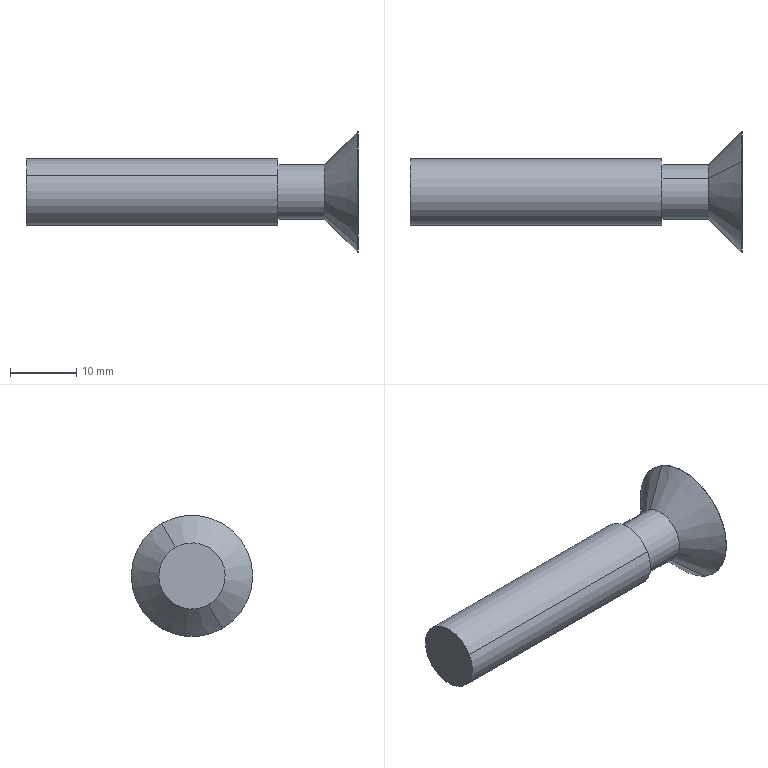Component | SolidWorks | CountersunkScrew-2 | 1 solid | 36 faces | box 50.07 x 18.3 x 18.3 mm | volume 3945 mm3 | plane 24 | cylinder 10 | cone 2 | commonest cylinder face diameters 4 x4 18.3 x2 8.3 x2 10 x2
STEP:
#1=COLOUR_RGB('',0.7922,0.8196,0.9333);
#2=FILL_AREA_STYLE_COLOUR('',#1);
#3=FILL_AREA_STYLE('',(#2));
#4=SURFACE_STYLE_FILL_AREA(#3);
#5=SURFACE_SIDE_STYLE('',(#4));
#6=SURFACE_STYLE_USAGE(.BOTH.,#5);
#7=PRESENTATION_STYLE_ASSIGNMENT((#6));
#8=CARTESIAN_POINT('',(2.939,29.846,46.096));
#9=VERTEX_POINT('',#8);
#10=CARTESIAN_POINT('',(2.939,30.206,46.72));
#11=VERTEX_POINT('',#10);
#12=CARTESIAN_POINT('',(2.939,30.026,46.408));
#13=DIRECTION('',(1.,0.,0.));
#14=DIRECTION('',(0.,-0.5,-0.866));
#15=AXIS2_PLACEMENT_3D('',#12,#13,#14);
#16=CIRCLE('',#15,0.3602);
#17=EDGE_CURVE('',#9,#11,#16,.T.);
#18=ORIENTED_EDGE('',*,*,#17,.F.);
#19=CARTESIAN_POINT('',(2.937,29.846,46.096));
#20=VERTEX_POINT('',#19);
#21=CARTESIAN_POINT('',(2.939,29.846,46.096));
#22=DIRECTION('',(-1.,0.,0.));
#23=VECTOR('',#22,39.37);
#24=LINE('',#21,#23);
#25=EDGE_CURVE('',#9,#20,#24,.T.);
#26=ORIENTED_EDGE('',*,*,#25,.T.);
#27=CARTESIAN_POINT('',(2.937,30.206,46.72));
#28=VERTEX_POINT('',#27);
#29=CARTESIAN_POINT('',(2.937,30.026,46.408));
#30=DIRECTION('',(1.,0.,0.));
#31=DIRECTION('',(0.,-0.5,-0.866));
#32=AXIS2_PLACEMENT_3D('',#29,#30,#31);
#33=CIRCLE('',#32,0.3602);
#34=EDGE_CURVE('',#20,#28,#33,.T.);
#35=ORIENTED_EDGE('',*,*,#34,.T.);
#36=CARTESIAN_POINT('',(2.939,30.206,46.72));
#37=DIRECTION('',(-1.,0.,0.));
#38=VECTOR('',#37,39.37);
#39=LINE('',#36,#38);
#40=EDGE_CURVE('',#11,#28,#39,.T.);
#41=ORIENTED_EDGE('',*,*,#40,.F.);
#42=EDGE_LOOP('',(#18,#26,#35,#41));
#43=FACE_OUTER_BOUND('',#42,.T.);
#44=CARTESIAN_POINT('',(2.939,30.026,46.408));
#45=DIRECTION('',(-1.,0.,0.));
#46=DIRECTION('',(0.,0.5,0.866));
#47=AXIS2_PLACEMENT_3D('',#44,#45,#46);
#48=CYLINDRICAL_SURFACE('',#47,0.3602);
#49=ADVANCED_FACE('',(#43),#48,.T.);
#50=CARTESIAN_POINT('',(2.74,29.945,46.266));
#51=VERTEX_POINT('',#50);
#52=CARTESIAN_POINT('',(2.74,30.108,46.549));
#53=VERTEX_POINT('',#52);
#54=CARTESIAN_POINT('',(2.74,30.026,46.408));
#55=DIRECTION('',(1.,0.,0.));
#56=DIRECTION('',(0.,-0.5,-0.866));
#57=AXIS2_PLACEMENT_3D('',#54,#55,#56);
#58=CIRCLE('',#57,0.1634);
#59=EDGE_CURVE('',#51,#53,#58,.T.);
#60=ORIENTED_EDGE('',*,*,#59,.T.);
#61=CARTESIAN_POINT('',(2.74,30.108,46.549));
#62=DIRECTION('',(0.7071,0.3536,0.6124));
#63=VECTOR('',#62,39.37);
#64=LINE('',#61,#63);
#65=EDGE_CURVE('',#53,#28,#64,.T.);
#66=ORIENTED_EDGE('',*,*,#65,.T.);
#67=ORIENTED_EDGE('',*,*,#34,.F.);
#68=CARTESIAN_POINT('',(2.74,29.945,46.266));
#69=DIRECTION('',(0.7071,-0.3536,-0.6124));
#70=VECTOR('',#69,39.37);
#71=LINE('',#68,#70);
#72=EDGE_CURVE('',#51,#20,#71,.T.);
#73=ORIENTED_EDGE('',*,*,#72,.F.);
#74=EDGE_LOOP('',(#60,#66,#67,#73));
#75=FACE_OUTER_BOUND('',#74,.T.);
#76=CARTESIAN_POINT('',(2.74,30.026,46.408));
#77=DIRECTION('',(1.,0.,0.));
#78=DIRECTION('',(0.,-0.5,-0.866));
#79=AXIS2_PLACEMENT_3D('',#76,#77,#78);
#80=CONICAL_SURFACE('',#79,0.1634,0.7854);
#81=ADVANCED_FACE('',(#75),#80,.T.);
#82=ORIENTED_EDGE('',*,*,#59,.F.);
#83=CARTESIAN_POINT('',(2.464,29.945,46.266));
#84=VERTEX_POINT('',#83);
#85=CARTESIAN_POINT('',(2.74,29.945,46.266));
#86=DIRECTION('',(-1.,0.,0.));
#87=VECTOR('',#86,39.37);
#88=LINE('',#85,#87);
#89=EDGE_CURVE('',#51,#84,#88,.T.);
#90=ORIENTED_EDGE('',*,*,#89,.T.);
#91=CARTESIAN_POINT('',(2.464,30.108,46.549));
#92=VERTEX_POINT('',#91);
#93=CARTESIAN_POINT('',(2.464,30.026,46.408));
#94=DIRECTION('',(1.,0.,0.));
#95=DIRECTION('',(0.,-0.5,-0.866));
#96=AXIS2_PLACEMENT_3D('',#93,#94,#95);
#97=CIRCLE('',#96,0.1634);
#98=EDGE_CURVE('',#84,#92,#97,.T.);
#99=ORIENTED_EDGE('',*,*,#98,.T.);
#100=CARTESIAN_POINT('',(2.74,30.108,46.549));
#101=DIRECTION('',(-1.,0.,0.));
#102=VECTOR('',#101,39.37);
#103=LINE('',#100,#102);
#104=EDGE_CURVE('',#53,#92,#103,.T.);
#105=ORIENTED_EDGE('',*,*,#104,.F.);
#106=EDGE_LOOP('',(#82,#90,#99,#105));
#107=FACE_OUTER_BOUND('',#106,.T.);
#108=CARTESIAN_POINT('',(2.74,30.026,46.408));
#109=DIRECTION('',(-1.,0.,0.));
#110=DIRECTION('',(0.,0.5,0.866));
#111=AXIS2_PLACEMENT_3D('',#108,#109,#110);
#112=CYLINDRICAL_SURFACE('',#111,0.1634);
#113=ADVANCED_FACE('',(#107),#112,.T.);
#114=CARTESIAN_POINT('',(2.464,30.197,46.309));
#115=VERTEX_POINT('',#114);
#116=CARTESIAN_POINT('',(2.464,29.856,46.506));
#117=VERTEX_POINT('',#116);
#118=CARTESIAN_POINT('',(2.464,30.026,46.408));
#119=DIRECTION('',(-1.,-0.,0.));
#120=DIRECTION('',(0.,0.866,-0.5));
#121=AXIS2_PLACEMENT_3D('',#118,#119,#120);
#122=CIRCLE('',#121,0.1969);
#123=EDGE_CURVE('',#115,#117,#122,.T.);
#124=ORIENTED_EDGE('',*,*,#123,.T.);
#125=CARTESIAN_POINT('',(0.9682,29.856,46.506));
#126=VERTEX_POINT('',#125);
#127=CARTESIAN_POINT('',(2.464,29.856,46.506));
#128=DIRECTION('',(-1.,-0.,0.));
#129=VECTOR('',#128,39.37);
#130=LINE('',#127,#129);
#131=EDGE_CURVE('',#117,#126,#130,.T.);
#132=ORIENTED_EDGE('',*,*,#131,.T.);
#133=CARTESIAN_POINT('',(0.9682,30.197,46.309));
#134=VERTEX_POINT('',#133);
#135=CARTESIAN_POINT('',(0.9682,30.026,46.408));
#136=DIRECTION('',(-1.,-0.,0.));
#137=DIRECTION('',(0.,0.866,-0.5));
#138=AXIS2_PLACEMENT_3D('',#135,#136,#137);
#139=CIRCLE('',#138,0.1969);
#140=EDGE_CURVE('',#134,#126,#139,.T.);
#141=ORIENTED_EDGE('',*,*,#140,.F.);
#142=CARTESIAN_POINT('',(2.464,30.197,46.309));
#143=DIRECTION('',(-1.,-0.,0.));
#144=VECTOR('',#143,39.37);
#145=LINE('',#142,#144);
#146=EDGE_CURVE('',#115,#134,#145,.T.);
#147=ORIENTED_EDGE('',*,*,#146,.F.);
#148=EDGE_LOOP('',(#124,#132,#141,#147));
#149=FACE_OUTER_BOUND('',#148,.T.);
#150=CARTESIAN_POINT('',(2.464,30.026,46.408));
#151=DIRECTION('',(-1.,-0.,0.));
#152=DIRECTION('',(0.,0.866,-0.5));
#153=AXIS2_PLACEMENT_3D('',#150,#151,#152);
#154=CYLINDRICAL_SURFACE('',#153,0.1969);
#155=ADVANCED_FACE('',(#149),#154,.T.);
#156=ORIENTED_EDGE('',*,*,#131,.F.);
#157=CARTESIAN_POINT('',(2.464,30.026,46.408));
#158=DIRECTION('',(-1.,-0.,0.));
#159=DIRECTION('',(0.,0.866,-0.5));
#160=AXIS2_PLACEMENT_3D('',#157,#158,#159);
#161=CIRCLE('',#160,0.1969);
#162=EDGE_CURVE('',#117,#115,#161,.T.);
#163=ORIENTED_EDGE('',*,*,#162,.T.);
#164=ORIENTED_EDGE('',*,*,#146,.T.);
#165=CARTESIAN_POINT('',(0.9682,30.026,46.408));
#166=DIRECTION('',(-1.,-0.,0.));
#167=DIRECTION('',(0.,0.866,-0.5));
#168=AXIS2_PLACEMENT_3D('',#165,#166,#167);
#169=CIRCLE('',#168,0.1969);
#170=EDGE_CURVE('',#126,#134,#169,.T.);
#171=ORIENTED_EDGE('',*,*,#170,.F.);
#172=EDGE_LOOP('',(#156,#163,#164,#171));
#173=FACE_OUTER_BOUND('',#172,.T.);
#174=CARTESIAN_POINT('',(2.464,30.026,46.408));
#175=DIRECTION('',(-1.,-0.,0.));
#176=DIRECTION('',(0.,0.866,-0.5));
#177=AXIS2_PLACEMENT_3D('',#174,#175,#176);
#178=CYLINDRICAL_SURFACE('',#177,0.1969);
#179=ADVANCED_FACE('',(#173),#178,.T.);
#180=CARTESIAN_POINT('',(2.464,30.026,46.408));
#181=DIRECTION('',(1.,0.,0.));
#182=DIRECTION('',(0.,-0.5,-0.866));
#183=AXIS2_PLACEMENT_3D('',#180,#181,#182);
#184=CIRCLE('',#183,0.1634);
#185=EDGE_CURVE('',#92,#84,#184,.T.);
#186=ORIENTED_EDGE('',*,*,#185,.F.);
#187=ORIENTED_EDGE('',*,*,#98,.F.);
#188=EDGE_LOOP('',(#186,#187));
#189=FACE_BOUND('',#188,.T.);
#190=ORIENTED_EDGE('',*,*,#123,.F.);
#191=ORIENTED_EDGE('',*,*,#162,.F.);
#192=EDGE_LOOP('',(#190,#191));
#193=FACE_OUTER_BOUND('',#192,.T.);
#194=CARTESIAN_POINT('',(2.464,29.928,46.237));
#195=DIRECTION('',(1.,0.,-0.));
#196=DIRECTION('',(0.,-0.866,0.5));
#197=AXIS2_PLACEMENT_3D('',#194,#195,#196);
#198=PLANE('',#197);
#199=ADVANCED_FACE('',(#189,#193),#198,.T.);
#200=ORIENTED_EDGE('',*,*,#140,.T.);
#201=ORIENTED_EDGE('',*,*,#170,.T.);
#202=EDGE_LOOP('',(#200,#201));
#203=FACE_OUTER_BOUND('',#202,.T.);
#204=CARTESIAN_POINT('',(0.9682,30.026,46.408));
#205=DIRECTION('',(-1.,-0.,0.));
#206=DIRECTION('',(-0.,0.866,-0.5));
#207=AXIS2_PLACEMENT_3D('',#204,#205,#206);
#208=PLANE('',#207);
#209=ADVANCED_FACE('',(#203),#208,.T.);
#210=ORIENTED_EDGE('',*,*,#89,.F.);
#211=CARTESIAN_POINT('',(2.74,30.026,46.408));
#212=DIRECTION('',(1.,0.,0.));
#213=DIRECTION('',(0.,-0.5,-0.866));
#214=AXIS2_PLACEMENT_3D('',#211,#212,#213);
#215=CIRCLE('',#214,0.1634);
#216=EDGE_CURVE('',#53,#51,#215,.T.);
#217=ORIENTED_EDGE('',*,*,#216,.F.);
#218=ORIENTED_EDGE('',*,*,#104,.T.);
#219=ORIENTED_EDGE('',*,*,#185,.T.);
#220=EDGE_LOOP('',(#210,#217,#218,#219));
#221=FACE_OUTER_BOUND('',#220,.T.);
#222=CARTESIAN_POINT('',(2.74,30.026,46.408));
#223=DIRECTION('',(-1.,0.,0.));
#224=DIRECTION('',(0.,0.5,0.866));
#225=AXIS2_PLACEMENT_3D('',#222,#223,#224);
#226=CYLINDRICAL_SURFACE('',#225,0.1634);
#227=ADVANCED_FACE('',(#221),#226,.T.);
#228=ORIENTED_EDGE('',*,*,#65,.F.);
#229=ORIENTED_EDGE('',*,*,#216,.T.);
#230=ORIENTED_EDGE('',*,*,#72,.T.);
#231=CARTESIAN_POINT('',(2.937,30.026,46.408));
#232=DIRECTION('',(1.,0.,0.));
#233=DIRECTION('',(0.,-0.5,-0.866));
#234=AXIS2_PLACEMENT_3D('',#231,#232,#233);
#235=CIRCLE('',#234,0.3602);
#236=EDGE_CURVE('',#28,#20,#235,.T.);
#237=ORIENTED_EDGE('',*,*,#236,.F.);
#238=EDGE_LOOP('',(#228,#229,#230,#237));
#239=FACE_OUTER_BOUND('',#238,.T.);
#240=CARTESIAN_POINT('',(2.74,30.026,46.408));
#241=DIRECTION('',(1.,0.,0.));
#242=DIRECTION('',(0.,-0.5,-0.866));
#243=AXIS2_PLACEMENT_3D('',#240,#241,#242);
#244=CONICAL_SURFACE('',#243,0.1634,0.7854);
#245=ADVANCED_FACE('',(#239),#244,.T.);
#246=ORIENTED_EDGE('',*,*,#25,.F.);
#247=CARTESIAN_POINT('',(2.939,30.026,46.408));
#248=DIRECTION('',(1.,0.,0.));
#249=DIRECTION('',(0.,-0.5,-0.866));
#250=AXIS2_PLACEMENT_3D('',#247,#248,#249);
#251=CIRCLE('',#250,0.3602);
#252=EDGE_CURVE('',#11,#9,#251,.T.);
#253=ORIENTED_EDGE('',*,*,#252,.F.);
#254=ORIENTED_EDGE('',*,*,#40,.T.);
#255=ORIENTED_EDGE('',*,*,#236,.T.);
#256=EDGE_LOOP('',(#246,#253,#254,#255));
#257=FACE_OUTER_BOUND('',#256,.T.);
#258=CARTESIAN_POINT('',(2.939,30.026,46.408));
#259=DIRECTION('',(-1.,0.,0.));
#260=DIRECTION('',(0.,0.5,0.866));
#261=AXIS2_PLACEMENT_3D('',#258,#259,#260);
#262=CYLINDRICAL_SURFACE('',#261,0.3602);
#263=ADVANCED_FACE('',(#257),#262,.T.);
#264=CARTESIAN_POINT('',(2.939,29.944,46.501));
#265=VERTEX_POINT('',#264);
#266=CARTESIAN_POINT('',(2.939,29.879,46.538));
#267=VERTEX_POINT('',#266);
#268=CARTESIAN_POINT('',(2.939,30.012,46.462));
#269=DIRECTION('',(0.,-0.866,0.5));
#270=VECTOR('',#269,39.37);
#271=LINE('',#268,#270);
#272=EDGE_CURVE('',#265,#267,#271,.T.);
#273=ORIENTED_EDGE('',*,*,#272,.F.);
#274=CARTESIAN_POINT('',(2.939,30.051,46.53));
#275=VERTEX_POINT('',#274);
#276=CARTESIAN_POINT('',(2.939,29.983,46.569));
#277=DIRECTION('',(1.,0.,0.));
#278=DIRECTION('',(0.,-0.5,-0.866));
#279=AXIS2_PLACEMENT_3D('',#276,#277,#278);
#280=CIRCLE('',#279,0.07874);
#281=EDGE_CURVE('',#265,#275,#280,.T.);
#282=ORIENTED_EDGE('',*,*,#281,.T.);
#283=CARTESIAN_POINT('',(2.939,30.089,46.595));
#284=VERTEX_POINT('',#283);
#285=CARTESIAN_POINT('',(2.939,30.032,46.496));
#286=DIRECTION('',(0.,-0.5,-0.866));
#287=VECTOR('',#286,39.37);
#288=LINE('',#285,#287);
#289=EDGE_CURVE('',#284,#275,#288,.T.);
#290=ORIENTED_EDGE('',*,*,#289,.F.);
#291=CARTESIAN_POINT('',(2.939,30.157,46.555));
#292=VERTEX_POINT('',#291);
#293=CARTESIAN_POINT('',(2.939,30.089,46.595));
#294=DIRECTION('',(0.,0.866,-0.5));
#295=VECTOR('',#294,39.37);
#296=LINE('',#293,#295);
#297=EDGE_CURVE('',#284,#292,#296,.T.);
#298=ORIENTED_EDGE('',*,*,#297,.T.);
#299=CARTESIAN_POINT('',(2.939,30.119,46.49));
#300=VERTEX_POINT('',#299);
#301=CARTESIAN_POINT('',(2.939,30.08,46.422));
#302=DIRECTION('',(0.,0.5,0.866));
#303=VECTOR('',#302,39.37);
#304=LINE('',#301,#303);
#305=EDGE_CURVE('',#300,#292,#304,.T.);
#306=ORIENTED_EDGE('',*,*,#305,.F.);
#307=CARTESIAN_POINT('',(2.939,30.148,46.383));
#308=VERTEX_POINT('',#307);
#309=CARTESIAN_POINT('',(2.939,30.188,46.451));
#310=DIRECTION('',(1.,0.,0.));
#311=DIRECTION('',(0.,-0.5,-0.866));
#312=AXIS2_PLACEMENT_3D('',#309,#310,#311);
#313=CIRCLE('',#312,0.07874);
#314=EDGE_CURVE('',#300,#308,#313,.T.);
#315=ORIENTED_EDGE('',*,*,#314,.T.);
#316=CARTESIAN_POINT('',(2.939,30.213,46.346));
#317=VERTEX_POINT('',#316);
#318=CARTESIAN_POINT('',(2.939,30.114,46.403));
#319=DIRECTION('',(0.,-0.866,0.5));
#320=VECTOR('',#319,39.37);
#321=LINE('',#318,#320);
#322=EDGE_CURVE('',#317,#308,#321,.T.);
#323=ORIENTED_EDGE('',*,*,#322,.F.);
#324=CARTESIAN_POINT('',(2.939,30.174,46.277));
#325=VERTEX_POINT('',#324);
#326=CARTESIAN_POINT('',(2.939,30.213,46.346));
#327=DIRECTION('',(0.,-0.5,-0.866));
#328=VECTOR('',#327,39.37);
#329=LINE('',#326,#328);
#330=EDGE_CURVE('',#317,#325,#329,.T.);
#331=ORIENTED_EDGE('',*,*,#330,.T.);
#332=CARTESIAN_POINT('',(2.939,30.109,46.315));
#333=VERTEX_POINT('',#332);
#334=CARTESIAN_POINT('',(2.939,30.041,46.354));
#335=DIRECTION('',(0.,0.866,-0.5));
#336=VECTOR('',#335,39.37);
#337=LINE('',#334,#336);
#338=EDGE_CURVE('',#333,#325,#337,.T.);
#339=ORIENTED_EDGE('',*,*,#338,.F.);
#340=CARTESIAN_POINT('',(2.939,30.001,46.286));
#341=VERTEX_POINT('',#340);
#342=CARTESIAN_POINT('',(2.939,30.069,46.247));
#343=DIRECTION('',(1.,0.,0.));
#344=DIRECTION('',(0.,-0.5,-0.866));
#345=AXIS2_PLACEMENT_3D('',#342,#343,#344);
#346=CIRCLE('',#345,0.07874);
#347=EDGE_CURVE('',#333,#341,#346,.T.);
#348=ORIENTED_EDGE('',*,*,#347,.T.);
#349=CARTESIAN_POINT('',(2.939,29.964,46.221));
#350=VERTEX_POINT('',#349);
#351=CARTESIAN_POINT('',(2.939,30.021,46.32));
#352=DIRECTION('',(0.,0.5,0.866));
#353=VECTOR('',#352,39.37);
#354=LINE('',#351,#353);
#355=EDGE_CURVE('',#350,#341,#354,.T.);
#356=ORIENTED_EDGE('',*,*,#355,.F.);
#357=CARTESIAN_POINT('',(2.939,29.896,46.26));
#358=VERTEX_POINT('',#357);
#359=CARTESIAN_POINT('',(2.939,29.964,46.221));
#360=DIRECTION('',(0.,-0.866,0.5));
#361=VECTOR('',#360,39.37);
#362=LINE('',#359,#361);
#363=EDGE_CURVE('',#350,#358,#362,.T.);
#364=ORIENTED_EDGE('',*,*,#363,.T.);
#365=CARTESIAN_POINT('',(2.939,29.933,46.325));
#366=VERTEX_POINT('',#365);
#367=CARTESIAN_POINT('',(2.939,29.972,46.393));
#368=DIRECTION('',(0.,-0.5,-0.866));
#369=VECTOR('',#368,39.37);
#370=LINE('',#367,#369);
#371=EDGE_CURVE('',#366,#358,#370,.T.);
#372=ORIENTED_EDGE('',*,*,#371,.F.);
#373=CARTESIAN_POINT('',(2.939,29.904,46.433));
#374=VERTEX_POINT('',#373);
#375=CARTESIAN_POINT('',(2.939,29.865,46.365));
#376=DIRECTION('',(1.,0.,0.));
#377=DIRECTION('',(0.,-0.5,-0.866));
#378=AXIS2_PLACEMENT_3D('',#375,#376,#377);
#379=CIRCLE('',#378,0.07874);
#380=EDGE_CURVE('',#366,#374,#379,.T.);
#381=ORIENTED_EDGE('',*,*,#380,.T.);
#382=CARTESIAN_POINT('',(2.939,29.84,46.47));
#383=VERTEX_POINT('',#382);
#384=CARTESIAN_POINT('',(2.939,29.938,46.413));
#385=DIRECTION('',(0.,0.866,-0.5));
#386=VECTOR('',#385,39.37);
#387=LINE('',#384,#386);
#388=EDGE_CURVE('',#383,#374,#387,.T.);
#389=ORIENTED_EDGE('',*,*,#388,.F.);
#390=CARTESIAN_POINT('',(2.939,29.84,46.47));
#391=DIRECTION('',(0.,0.5,0.866));
#392=VECTOR('',#391,39.37);
#393=LINE('',#390,#392);
#394=EDGE_CURVE('',#383,#267,#393,.T.);
#395=ORIENTED_EDGE('',*,*,#394,.T.);
#396=EDGE_LOOP('',(#273,#282,#290,#298,#306,#315,#323,#331,#339,#348,#356,#364,#372,#381,#389,#395));
#397=FACE_BOUND('',#396,.T.);
#398=ORIENTED_EDGE('',*,*,#252,.T.);
#399=ORIENTED_EDGE('',*,*,#17,.T.);
#400=EDGE_LOOP('',(#398,#399));
#401=FACE_OUTER_BOUND('',#400,.T.);
#402=CARTESIAN_POINT('',(2.939,30.026,46.408));
#403=DIRECTION('',(1.,0.,0.));
#404=DIRECTION('',(0.,-0.5,-0.866));
#405=AXIS2_PLACEMENT_3D('',#402,#403,#404);
#406=PLANE('',#405);
#407=ADVANCED_FACE('',(#397,#401),#406,.T.);
#408=CARTESIAN_POINT('',(2.717,29.983,46.49));
#409=VERTEX_POINT('',#408);
#410=CARTESIAN_POINT('',(2.717,29.933,46.404));
#411=VERTEX_POINT('',#410);
#412=CARTESIAN_POINT('',(2.717,29.978,46.481));
#413=DIRECTION('',(0.,-0.5,-0.866));
#414=VECTOR('',#413,39.37);
#415=LINE('',#412,#414);
#416=EDGE_CURVE('',#409,#411,#415,.T.);
#417=ORIENTED_EDGE('',*,*,#416,.F.);
#418=CARTESIAN_POINT('',(2.755,29.983,46.49));
#419=VERTEX_POINT('',#418);
#420=CARTESIAN_POINT('',(2.717,29.983,46.49));
#421=DIRECTION('',(1.,0.,0.));
#422=VECTOR('',#421,39.37);
#423=LINE('',#420,#422);
#424=EDGE_CURVE('',#409,#419,#423,.T.);
#425=ORIENTED_EDGE('',*,*,#424,.T.);
#426=CARTESIAN_POINT('',(2.755,29.933,46.404));
#427=VERTEX_POINT('',#426);
#428=CARTESIAN_POINT('',(2.755,29.978,46.481));
#429=DIRECTION('',(0.,-0.5,-0.866));
#430=VECTOR('',#429,39.37);
#431=LINE('',#428,#430);
#432=EDGE_CURVE('',#419,#427,#431,.T.);
#433=ORIENTED_EDGE('',*,*,#432,.T.);
#434=CARTESIAN_POINT('',(2.755,29.933,46.404));
#435=DIRECTION('',(-1.,0.,0.));
#436=VECTOR('',#435,39.37);
#437=LINE('',#434,#436);
#438=EDGE_CURVE('',#427,#411,#437,.T.);
#439=ORIENTED_EDGE('',*,*,#438,.T.);
#440=EDGE_LOOP('',(#417,#425,#433,#439));
#441=FACE_OUTER_BOUND('',#440,.T.);
#442=CARTESIAN_POINT('',(2.717,29.978,46.481));
#443=DIRECTION('',(0.,-0.866,0.5));
#444=DIRECTION('',(-1.,0.,0.));
#445=AXIS2_PLACEMENT_3D('',#442,#443,#444);
#446=PLANE('',#445);
#447=ADVANCED_FACE('',(#441),#446,.F.);
#448=CARTESIAN_POINT('',(2.865,29.879,46.538));
#449=VERTEX_POINT('',#448);
#450=CARTESIAN_POINT('',(2.793,29.944,46.501));
#451=VERTEX_POINT('',#450);
#452=CARTESIAN_POINT('',(2.865,29.879,46.538));
#453=DIRECTION('',(-0.6941,0.6235,-0.36));
#454=VECTOR('',#453,39.37);
#455=LINE('',#452,#454);
#456=EDGE_CURVE('',#449,#451,#455,.T.);
#457=ORIENTED_EDGE('',*,*,#456,.T.);
#458=CARTESIAN_POINT('',(2.717,29.944,46.501));
#459=DIRECTION('',(1.,0.,0.));
#460=VECTOR('',#459,39.37);
#461=LINE('',#458,#460);
#462=EDGE_CURVE('',#451,#265,#461,.T.);
#463=ORIENTED_EDGE('',*,*,#462,.T.);
#464=ORIENTED_EDGE('',*,*,#272,.T.);
#465=CARTESIAN_POINT('',(3.078,29.879,46.538));
#466=DIRECTION('',(-1.,0.,0.));
#467=VECTOR('',#466,39.37);
#468=LINE('',#465,#467);
#469=EDGE_CURVE('',#267,#449,#468,.T.);
#470=ORIENTED_EDGE('',*,*,#469,.T.);
#471=EDGE_LOOP('',(#457,#463,#464,#470));
#472=FACE_OUTER_BOUND('',#471,.T.);
#473=CARTESIAN_POINT('',(2.717,30.012,46.462));
#474=DIRECTION('',(0.,0.5,0.866));
#475=DIRECTION('',(1.,0.,0.));
#476=AXIS2_PLACEMENT_3D('',#473,#474,#475);
#477=PLANE('',#476);
#478=ADVANCED_FACE('',(#472),#477,.F.);
#479=ORIENTED_EDGE('',*,*,#289,.T.);
#480=CARTESIAN_POINT('',(2.793,30.051,46.53));
#481=VERTEX_POINT('',#480);
#482=CARTESIAN_POINT('',(2.717,30.051,46.53));
#483=DIRECTION('',(-1.,0.,0.));
#484=VECTOR('',#483,39.37);
#485=LINE('',#482,#484);
#486=EDGE_CURVE('',#275,#481,#485,.T.);
#487=ORIENTED_EDGE('',*,*,#486,.T.);
#488=CARTESIAN_POINT('',(2.865,30.089,46.595));
#489=VERTEX_POINT('',#488);
#490=CARTESIAN_POINT('',(2.865,30.089,46.595));
#491=DIRECTION('',(0.6941,0.36,0.6235));
#492=VECTOR('',#491,39.37);
#493=LINE('',#490,#492);
#494=EDGE_CURVE('',#481,#489,#493,.T.);
#495=ORIENTED_EDGE('',*,*,#494,.T.);
#496=CARTESIAN_POINT('',(3.078,30.089,46.595));
#497=DIRECTION('',(-1.,0.,0.));
#498=VECTOR('',#497,39.37);
#499=LINE('',#496,#498);
#500=EDGE_CURVE('',#284,#489,#499,.T.);
#501=ORIENTED_EDGE('',*,*,#500,.F.);
#502=EDGE_LOOP('',(#479,#487,#495,#501));
#503=FACE_OUTER_BOUND('',#502,.T.);
#504=CARTESIAN_POINT('',(2.717,30.032,46.496));
#505=DIRECTION('',(0.,-0.866,0.5));
#506=DIRECTION('',(-1.,0.,0.));
#507=AXIS2_PLACEMENT_3D('',#504,#505,#506);
#508=PLANE('',#507);
#509=ADVANCED_FACE('',(#503),#508,.F.);
#510=CARTESIAN_POINT('',(2.717,30.109,46.451));
#511=VERTEX_POINT('',#510);
#512=CARTESIAN_POINT('',(2.717,30.022,46.501));
#513=VERTEX_POINT('',#512);
#514=CARTESIAN_POINT('',(2.717,30.1,46.456));
#515=DIRECTION('',(0.,-0.866,0.5));
#516=VECTOR('',#515,39.37);
#517=LINE('',#514,#516);
#518=EDGE_CURVE('',#511,#513,#517,.T.);
#519=ORIENTED_EDGE('',*,*,#518,.F.);
#520=CARTESIAN_POINT('',(2.755,30.109,46.451));
#521=VERTEX_POINT('',#520);
#522=CARTESIAN_POINT('',(2.717,30.109,46.451));
#523=DIRECTION('',(1.,0.,0.));
#524=VECTOR('',#523,39.37);
#525=LINE('',#522,#524);
#526=EDGE_CURVE('',#511,#521,#525,.T.);
#527=ORIENTED_EDGE('',*,*,#526,.T.);
#528=CARTESIAN_POINT('',(2.755,30.022,46.501));
#529=VERTEX_POINT('',#528);
#530=CARTESIAN_POINT('',(2.755,30.1,46.456));
#531=DIRECTION('',(0.,-0.866,0.5));
#532=VECTOR('',#531,39.37);
#533=LINE('',#530,#532);
#534=EDGE_CURVE('',#521,#529,#533,.T.);
#535=ORIENTED_EDGE('',*,*,#534,.T.);
#536=CARTESIAN_POINT('',(2.755,30.022,46.501));
#537=DIRECTION('',(-1.,0.,0.));
#538=VECTOR('',#537,39.37);
#539=LINE('',#536,#538);
#540=EDGE_CURVE('',#529,#513,#539,.T.);
#541=ORIENTED_EDGE('',*,*,#540,.T.);
#542=EDGE_LOOP('',(#519,#527,#535,#541));
#543=FACE_OUTER_BOUND('',#542,.T.);
#544=CARTESIAN_POINT('',(2.717,30.1,46.456));
#545=DIRECTION('',(0.,0.5,0.866));
#546=DIRECTION('',(1.,0.,0.));
#547=AXIS2_PLACEMENT_3D('',#544,#545,#546);
#548=PLANE('',#547);
#549=ADVANCED_FACE('',(#543),#548,.F.);
#550=CARTESIAN_POINT('',(2.865,30.157,46.555));
#551=VERTEX_POINT('',#550);
#552=CARTESIAN_POINT('',(2.793,30.119,46.49));
#553=VERTEX_POINT('',#552);
#554=CARTESIAN_POINT('',(2.865,30.157,46.555));
#555=DIRECTION('',(-0.6941,-0.36,-0.6235));
#556=VECTOR('',#555,39.37);
#557=LINE('',#554,#556);
#558=EDGE_CURVE('',#551,#553,#557,.T.);
#559=ORIENTED_EDGE('',*,*,#558,.T.);
#560=CARTESIAN_POINT('',(2.717,30.119,46.49));
#561=DIRECTION('',(1.,0.,0.));
#562=VECTOR('',#561,39.37);
#563=LINE('',#560,#562);
#564=EDGE_CURVE('',#553,#300,#563,.T.);
#565=ORIENTED_EDGE('',*,*,#564,.T.);
#566=ORIENTED_EDGE('',*,*,#305,.T.);
#567=CARTESIAN_POINT('',(3.078,30.157,46.555));
#568=DIRECTION('',(-1.,0.,0.));
#569=VECTOR('',#568,39.37);
#570=LINE('',#567,#569);
#571=EDGE_CURVE('',#292,#551,#570,.T.);
#572=ORIENTED_EDGE('',*,*,#571,.T.);
#573=EDGE_LOOP('',(#559,#565,#566,#572));
#574=FACE_OUTER_BOUND('',#573,.T.);
#575=CARTESIAN_POINT('',(2.717,30.08,46.422));
#576=DIRECTION('',(0.,0.866,-0.5));
#577=DIRECTION('',(1.,0.,0.));
#578=AXIS2_PLACEMENT_3D('',#575,#576,#577);
#579=PLANE('',#578);
#580=ADVANCED_FACE('',(#574),#579,.F.);
#581=ORIENTED_EDGE('',*,*,#322,.T.);
#582=CARTESIAN_POINT('',(2.793,30.148,46.383));
#583=VERTEX_POINT('',#582);
#584=CARTESIAN_POINT('',(2.717,30.148,46.383));
#585=DIRECTION('',(-1.,0.,0.));
#586=VECTOR('',#585,39.37);
#587=LINE('',#584,#586);
#588=EDGE_CURVE('',#308,#583,#587,.T.);
#589=ORIENTED_EDGE('',*,*,#588,.T.);
#590=CARTESIAN_POINT('',(2.865,30.213,46.346));
#591=VERTEX_POINT('',#590);
#592=CARTESIAN_POINT('',(2.865,30.213,46.346));
#593=DIRECTION('',(0.6941,0.6235,-0.36));
#594=VECTOR('',#593,39.37);
#595=LINE('',#592,#594);
#596=EDGE_CURVE('',#583,#591,#595,.T.);
#597=ORIENTED_EDGE('',*,*,#596,.T.);
#598=CARTESIAN_POINT('',(3.078,30.213,46.346));
#599=DIRECTION('',(-1.,0.,0.));
#600=VECTOR('',#599,39.37);
#601=LINE('',#598,#600);
#602=EDGE_CURVE('',#317,#591,#601,.T.);
#603=ORIENTED_EDGE('',*,*,#602,.F.);
#604=EDGE_LOOP('',(#581,#589,#597,#603));
#605=FACE_OUTER_BOUND('',#604,.T.);
#606=CARTESIAN_POINT('',(2.717,30.114,46.403));
#607=DIRECTION('',(0.,0.5,0.866));
#608=DIRECTION('',(0.,-0.866,0.5));
#609=AXIS2_PLACEMENT_3D('',#606,#607,#608);
#610=PLANE('',#609);
#611=ADVANCED_FACE('',(#605),#610,.F.);
#612=CARTESIAN_POINT('',(2.717,30.069,46.325));
#613=VERTEX_POINT('',#612);
#614=CARTESIAN_POINT('',(2.717,30.119,46.412));
#615=VERTEX_POINT('',#614);
#616=CARTESIAN_POINT('',(2.717,30.075,46.334));
#617=DIRECTION('',(0.,0.5,0.866));
#618=VECTOR('',#617,39.37);
#619=LINE('',#616,#618);
#620=EDGE_CURVE('',#613,#615,#619,.T.);
#621=ORIENTED_EDGE('',*,*,#620,.F.);
#622=CARTESIAN_POINT('',(2.755,30.069,46.325));
#623=VERTEX_POINT('',#622);
#624=CARTESIAN_POINT('',(2.717,30.069,46.325));
#625=DIRECTION('',(1.,0.,0.));
#626=VECTOR('',#625,39.37);
#627=LINE('',#624,#626);
#628=EDGE_CURVE('',#613,#623,#627,.T.);
#629=ORIENTED_EDGE('',*,*,#628,.T.);
#630=CARTESIAN_POINT('',(2.755,30.119,46.412));
#631=VERTEX_POINT('',#630);
#632=CARTESIAN_POINT('',(2.755,30.075,46.334));
#633=DIRECTION('',(0.,0.5,0.866));
#634=VECTOR('',#633,39.37);
#635=LINE('',#632,#634);
#636=EDGE_CURVE('',#623,#631,#635,.T.);
#637=ORIENTED_EDGE('',*,*,#636,.T.);
#638=CARTESIAN_POINT('',(2.755,30.119,46.412));
#639=DIRECTION('',(-1.,0.,0.));
#640=VECTOR('',#639,39.37);
#641=LINE('',#638,#640);
#642=EDGE_CURVE('',#631,#615,#641,.T.);
#643=ORIENTED_EDGE('',*,*,#642,.T.);
#644=EDGE_LOOP('',(#621,#629,#637,#643));
#645=FACE_OUTER_BOUND('',#644,.T.);
#646=CARTESIAN_POINT('',(2.717,30.075,46.334));
#647=DIRECTION('',(0.,0.866,-0.5));
#648=DIRECTION('',(1.,0.,0.));
#649=AXIS2_PLACEMENT_3D('',#646,#647,#648);
#650=PLANE('',#649);
#651=ADVANCED_FACE('',(#645),#650,.F.);
#652=CARTESIAN_POINT('',(2.865,30.174,46.277));
#653=VERTEX_POINT('',#652);
#654=CARTESIAN_POINT('',(2.793,30.109,46.315));
#655=VERTEX_POINT('',#654);
#656=CARTESIAN_POINT('',(2.865,30.174,46.277));
#657=DIRECTION('',(-0.6941,-0.6235,0.36));
#658=VECTOR('',#657,39.37);
#659=LINE('',#656,#658);
#660=EDGE_CURVE('',#653,#655,#659,.T.);
#661=ORIENTED_EDGE('',*,*,#660,.T.);
#662=CARTESIAN_POINT('',(2.717,30.109,46.315));
#663=DIRECTION('',(1.,0.,0.));
#664=VECTOR('',#663,39.37);
#665=LINE('',#662,#664);
#666=EDGE_CURVE('',#655,#333,#665,.T.);
#667=ORIENTED_EDGE('',*,*,#666,.T.);
#668=ORIENTED_EDGE('',*,*,#338,.T.);
#669=CARTESIAN_POINT('',(3.078,30.174,46.277));
#670=DIRECTION('',(-1.,0.,0.));
#671=VECTOR('',#670,39.37);
#672=LINE('',#669,#671);
#673=EDGE_CURVE('',#325,#653,#672,.T.);
#674=ORIENTED_EDGE('',*,*,#673,.T.);
#675=EDGE_LOOP('',(#661,#667,#668,#674));
#676=FACE_OUTER_BOUND('',#675,.T.);
#677=CARTESIAN_POINT('',(2.717,30.041,46.354));
#678=DIRECTION('',(0.,-0.5,-0.866));
#679=DIRECTION('',(-1.,0.,0.));
#680=AXIS2_PLACEMENT_3D('',#677,#678,#679);
#681=PLANE('',#680);
#682=ADVANCED_FACE('',(#676),#681,.F.);
#683=ORIENTED_EDGE('',*,*,#355,.T.);
#684=CARTESIAN_POINT('',(2.793,30.001,46.286));
#685=VERTEX_POINT('',#684);
#686=CARTESIAN_POINT('',(2.717,30.001,46.286));
#687=DIRECTION('',(-1.,0.,0.));
#688=VECTOR('',#687,39.37);
#689=LINE('',#686,#688);
#690=EDGE_CURVE('',#341,#685,#689,.T.);
#691=ORIENTED_EDGE('',*,*,#690,.T.);
#692=CARTESIAN_POINT('',(2.865,29.964,46.221));
#693=VERTEX_POINT('',#692);
#694=CARTESIAN_POINT('',(2.865,29.964,46.221));
#695=DIRECTION('',(0.6941,-0.36,-0.6235));
#696=VECTOR('',#695,39.37);
#697=LINE('',#694,#696);
#698=EDGE_CURVE('',#685,#693,#697,.T.);
#699=ORIENTED_EDGE('',*,*,#698,.T.);
#700=CARTESIAN_POINT('',(3.078,29.964,46.221));
#701=DIRECTION('',(-1.,0.,0.));
#702=VECTOR('',#701,39.37);
#703=LINE('',#700,#702);
#704=EDGE_CURVE('',#350,#693,#703,.T.);
#705=ORIENTED_EDGE('',*,*,#704,.F.);
#706=EDGE_LOOP('',(#683,#691,#699,#705));
#707=FACE_OUTER_BOUND('',#706,.T.);
#708=CARTESIAN_POINT('',(2.717,30.021,46.32));
#709=DIRECTION('',(0.,0.866,-0.5));
#710=DIRECTION('',(1.,0.,0.));
#711=AXIS2_PLACEMENT_3D('',#708,#709,#710);
#712=PLANE('',#711);
#713=ADVANCED_FACE('',(#707),#712,.F.);
#714=CARTESIAN_POINT('',(2.717,29.944,46.365));
#715=VERTEX_POINT('',#714);
#716=CARTESIAN_POINT('',(2.717,30.03,46.315));
#717=VERTEX_POINT('',#716);
#718=CARTESIAN_POINT('',(2.717,29.953,46.359));
#719=DIRECTION('',(0.,0.866,-0.5));
#720=VECTOR('',#719,39.37);
#721=LINE('',#718,#720);
#722=EDGE_CURVE('',#715,#717,#721,.T.);
#723=ORIENTED_EDGE('',*,*,#722,.F.);
#724=CARTESIAN_POINT('',(2.755,29.944,46.365));
#725=VERTEX_POINT('',#724);
#726=CARTESIAN_POINT('',(2.717,29.944,46.365));
#727=DIRECTION('',(1.,0.,0.));
#728=VECTOR('',#727,39.37);
#729=LINE('',#726,#728);
#730=EDGE_CURVE('',#715,#725,#729,.T.);
#731=ORIENTED_EDGE('',*,*,#730,.T.);
#732=CARTESIAN_POINT('',(2.755,30.03,46.315));
#733=VERTEX_POINT('',#732);
#734=CARTESIAN_POINT('',(2.755,29.953,46.359));
#735=DIRECTION('',(0.,0.866,-0.5));
#736=VECTOR('',#735,39.37);
#737=LINE('',#734,#736);
#738=EDGE_CURVE('',#725,#733,#737,.T.);
#739=ORIENTED_EDGE('',*,*,#738,.T.);
#740=CARTESIAN_POINT('',(2.755,30.03,46.315));
#741=DIRECTION('',(-1.,0.,0.));
#742=VECTOR('',#741,39.37);
#743=LINE('',#740,#742);
#744=EDGE_CURVE('',#733,#717,#743,.T.);
#745=ORIENTED_EDGE('',*,*,#744,.T.);
#746=EDGE_LOOP('',(#723,#731,#739,#745));
#747=FACE_OUTER_BOUND('',#746,.T.);
#748=CARTESIAN_POINT('',(2.717,29.953,46.359));
#749=DIRECTION('',(0.,-0.5,-0.866));
#750=DIRECTION('',(-1.,0.,0.));
#751=AXIS2_PLACEMENT_3D('',#748,#749,#750);
#752=PLANE('',#751);
#753=ADVANCED_FACE('',(#747),#752,.F.);
#754=CARTESIAN_POINT('',(2.865,29.896,46.26));
#755=VERTEX_POINT('',#754);
#756=CARTESIAN_POINT('',(2.793,29.933,46.325));
#757=VERTEX_POINT('',#756);
#758=CARTESIAN_POINT('',(2.865,29.896,46.26));
#759=DIRECTION('',(-0.6941,0.36,0.6235));
#760=VECTOR('',#759,39.37);
#761=LINE('',#758,#760);
#762=EDGE_CURVE('',#755,#757,#761,.T.);
#763=ORIENTED_EDGE('',*,*,#762,.T.);
#764=CARTESIAN_POINT('',(2.717,29.933,46.325));
#765=DIRECTION('',(1.,0.,0.));
#766=VECTOR('',#765,39.37);
#767=LINE('',#764,#766);
#768=EDGE_CURVE('',#757,#366,#767,.T.);
#769=ORIENTED_EDGE('',*,*,#768,.T.);
#770=ORIENTED_EDGE('',*,*,#371,.T.);
#771=CARTESIAN_POINT('',(3.078,29.896,46.26));
#772=DIRECTION('',(-1.,0.,0.));
#773=VECTOR('',#772,39.37);
#774=LINE('',#771,#773);
#775=EDGE_CURVE('',#358,#755,#774,.T.);
#776=ORIENTED_EDGE('',*,*,#775,.T.);
#777=EDGE_LOOP('',(#763,#769,#770,#776));
#778=FACE_OUTER_BOUND('',#777,.T.);
#779=CARTESIAN_POINT('',(2.717,29.972,46.393));
#780=DIRECTION('',(0.,-0.866,0.5));
#781=DIRECTION('',(-1.,0.,0.));
#782=AXIS2_PLACEMENT_3D('',#779,#780,#781);
#783=PLANE('',#782);
#784=ADVANCED_FACE('',(#778),#783,.F.);
#785=ORIENTED_EDGE('',*,*,#388,.T.);
#786=CARTESIAN_POINT('',(2.793,29.904,46.433));
#787=VERTEX_POINT('',#786);
#788=CARTESIAN_POINT('',(2.717,29.904,46.433));
#789=DIRECTION('',(-1.,0.,0.));
#790=VECTOR('',#789,39.37);
#791=LINE('',#788,#790);
#792=EDGE_CURVE('',#374,#787,#791,.T.);
#793=ORIENTED_EDGE('',*,*,#792,.T.);
#794=CARTESIAN_POINT('',(2.865,29.84,46.47));
#795=VERTEX_POINT('',#794);
#796=CARTESIAN_POINT('',(2.865,29.84,46.47));
#797=DIRECTION('',(0.6941,-0.6235,0.36));
#798=VECTOR('',#797,39.37);
#799=LINE('',#796,#798);
#800=EDGE_CURVE('',#787,#795,#799,.T.);
#801=ORIENTED_EDGE('',*,*,#800,.T.);
#802=CARTESIAN_POINT('',(3.078,29.84,46.47));
#803=DIRECTION('',(-1.,0.,0.));
#804=VECTOR('',#803,39.37);
#805=LINE('',#802,#804);
#806=EDGE_CURVE('',#383,#795,#805,.T.);
#807=ORIENTED_EDGE('',*,*,#806,.F.);
#808=EDGE_LOOP('',(#785,#793,#801,#807));
#809=FACE_OUTER_BOUND('',#808,.T.);
#810=CARTESIAN_POINT('',(2.717,29.938,46.413));
#811=DIRECTION('',(0.,-0.5,-0.866));
#812=DIRECTION('',(-1.,0.,0.));
#813=AXIS2_PLACEMENT_3D('',#810,#811,#812);
#814=PLANE('',#813);
#815=ADVANCED_FACE('',(#809),#814,.F.);
#816=ORIENTED_EDGE('',*,*,#416,.T.);
#817=CARTESIAN_POINT('',(2.717,29.865,46.365));
#818=DIRECTION('',(-1.,0.,0.));
#819=DIRECTION('',(0.,-0.5,-0.866));
#820=AXIS2_PLACEMENT_3D('',#817,#818,#819);
#821=CIRCLE('',#820,0.07874);
#822=EDGE_CURVE('',#411,#715,#821,.T.);
#823=ORIENTED_EDGE('',*,*,#822,.T.);
#824=ORIENTED_EDGE('',*,*,#722,.T.);
#825=CARTESIAN_POINT('',(2.717,30.069,46.247));
#826=DIRECTION('',(-1.,0.,0.));
#827=DIRECTION('',(0.,-0.5,-0.866));
#828=AXIS2_PLACEMENT_3D('',#825,#826,#827);
#829=CIRCLE('',#828,0.07874);
#830=EDGE_CURVE('',#717,#613,#829,.T.);
#831=ORIENTED_EDGE('',*,*,#830,.T.);
#832=ORIENTED_EDGE('',*,*,#620,.T.);
#833=CARTESIAN_POINT('',(2.717,30.188,46.451));
#834=DIRECTION('',(-1.,0.,0.));
#835=DIRECTION('',(0.,-0.5,-0.866));
#836=AXIS2_PLACEMENT_3D('',#833,#834,#835);
#837=CIRCLE('',#836,0.07874);
#838=EDGE_CURVE('',#615,#511,#837,.T.);
#839=ORIENTED_EDGE('',*,*,#838,.T.);
#840=ORIENTED_EDGE('',*,*,#518,.T.);
#841=CARTESIAN_POINT('',(2.717,29.983,46.569));
#842=DIRECTION('',(-1.,0.,0.));
#843=DIRECTION('',(0.,-0.5,-0.866));
#844=AXIS2_PLACEMENT_3D('',#841,#842,#843);
#845=CIRCLE('',#844,0.07874);
#846=EDGE_CURVE('',#513,#409,#845,.T.);
#847=ORIENTED_EDGE('',*,*,#846,.T.);
#848=EDGE_LOOP('',(#816,#823,#824,#831,#832,#839,#840,#847));
#849=FACE_OUTER_BOUND('',#848,.T.);
#850=CARTESIAN_POINT('',(2.717,30.026,46.408));
#851=DIRECTION('',(1.,0.,0.));
#852=DIRECTION('',(0.,-0.5,-0.866));
#853=AXIS2_PLACEMENT_3D('',#850,#851,#852);
#854=PLANE('',#853);
#855=ADVANCED_FACE('',(#849),#854,.T.);
#856=ORIENTED_EDGE('',*,*,#534,.F.);
#857=CARTESIAN_POINT('',(2.755,30.109,46.451));
#858=CARTESIAN_POINT('',(2.767,30.109,46.465));
#859=CARTESIAN_POINT('',(2.78,30.112,46.478));
#860=CARTESIAN_POINT('',(2.793,30.119,46.49));
#861=(BOUNDED_CURVE()B_SPLINE_CURVE(3,(#857,#858,#859,#860),.UNSPECIFIED.,.F.,.T.)B_SPLINE_CURVE_WITH_KNOTS((4,4),(4.189,4.712),.UNSPECIFIED.)CURVE()GEOMETRIC_REPRESENTATION_ITEM()RATIONAL_B_SPLINE_CURVE((1.,0.9773,0.9773,1.))REPRESENTATION_ITEM(''));
#862=EDGE_CURVE('',#521,#553,#861,.T.);
#863=ORIENTED_EDGE('',*,*,#862,.T.);
#864=ORIENTED_EDGE('',*,*,#558,.F.);
#865=CARTESIAN_POINT('',(2.865,30.089,46.595));
#866=DIRECTION('',(0.,0.866,-0.5));
#867=VECTOR('',#866,39.37);
#868=LINE('',#865,#867);
#869=EDGE_CURVE('',#489,#551,#868,.T.);
#870=ORIENTED_EDGE('',*,*,#869,.F.);
#871=ORIENTED_EDGE('',*,*,#494,.F.);
#872=CARTESIAN_POINT('',(2.793,30.051,46.53));
#873=CARTESIAN_POINT('',(2.78,30.044,46.518));
#874=CARTESIAN_POINT('',(2.767,30.034,46.508));
#875=CARTESIAN_POINT('',(2.755,30.022,46.501));
#876=(BOUNDED_CURVE()B_SPLINE_CURVE(3,(#872,#873,#874,#875),.UNSPECIFIED.,.F.,.F.)B_SPLINE_CURVE_WITH_KNOTS((4,4),(1.571,2.094),.UNSPECIFIED.)CURVE()GEOMETRIC_REPRESENTATION_ITEM()RATIONAL_B_SPLINE_CURVE((1.,0.9773,0.9773,1.))REPRESENTATION_ITEM(''));
#877=EDGE_CURVE('',#481,#529,#876,.T.);
#878=ORIENTED_EDGE('',*,*,#877,.T.);
#879=EDGE_LOOP('',(#856,#863,#864,#870,#871,#878));
#880=FACE_OUTER_BOUND('',#879,.T.);
#881=CARTESIAN_POINT('',(2.865,30.089,46.595));
#882=DIRECTION('',(0.7199,-0.347,-0.6011));
#883=DIRECTION('',(-0.6941,-0.36,-0.6235));
#884=AXIS2_PLACEMENT_3D('',#881,#882,#883);
#885=PLANE('',#884);
#886=ADVANCED_FACE('',(#880),#885,.T.);
#887=ORIENTED_EDGE('',*,*,#500,.T.);
#888=ORIENTED_EDGE('',*,*,#869,.T.);
#889=ORIENTED_EDGE('',*,*,#571,.F.);
#890=ORIENTED_EDGE('',*,*,#297,.F.);
#891=EDGE_LOOP('',(#887,#888,#889,#890));
#892=FACE_OUTER_BOUND('',#891,.T.);
#893=CARTESIAN_POINT('',(3.078,30.089,46.595));
#894=DIRECTION('',(0.,0.5,0.866));
#895=DIRECTION('',(1.,0.,0.));
#896=AXIS2_PLACEMENT_3D('',#893,#894,#895);
#897=PLANE('',#896);
#898=ADVANCED_FACE('',(#892),#897,.F.);
#899=ORIENTED_EDGE('',*,*,#636,.F.);
#900=CARTESIAN_POINT('',(2.755,30.069,46.325));
#901=CARTESIAN_POINT('',(2.767,30.083,46.325));
#902=CARTESIAN_POINT('',(2.78,30.097,46.322));
#903=CARTESIAN_POINT('',(2.793,30.109,46.315));
#904=(BOUNDED_CURVE()B_SPLINE_CURVE(3,(#900,#901,#902,#903),.UNSPECIFIED.,.F.,.F.)B_SPLINE_CURVE_WITH_KNOTS((4,4),(4.189,4.712),.UNSPECIFIED.)CURVE()GEOMETRIC_REPRESENTATION_ITEM()RATIONAL_B_SPLINE_CURVE((1.,0.9773,0.9773,1.))REPRESENTATION_ITEM(''));
#905=EDGE_CURVE('',#623,#655,#904,.T.);
#906=ORIENTED_EDGE('',*,*,#905,.T.);
#907=ORIENTED_EDGE('',*,*,#660,.F.);
#908=CARTESIAN_POINT('',(2.865,30.213,46.346));
#909=DIRECTION('',(0.,-0.5,-0.866));
#910=VECTOR('',#909,39.37);
#911=LINE('',#908,#910);
#912=EDGE_CURVE('',#591,#653,#911,.T.);
#913=ORIENTED_EDGE('',*,*,#912,.F.);
#914=ORIENTED_EDGE('',*,*,#596,.F.);
#915=CARTESIAN_POINT('',(2.793,30.148,46.383));
#916=CARTESIAN_POINT('',(2.78,30.136,46.39));
#917=CARTESIAN_POINT('',(2.767,30.126,46.4));
#918=CARTESIAN_POINT('',(2.755,30.119,46.412));
#919=(BOUNDED_CURVE()B_SPLINE_CURVE(3,(#915,#916,#917,#918),.UNSPECIFIED.,.F.,.F.)B_SPLINE_CURVE_WITH_KNOTS((4,4),(1.571,2.094),.UNSPECIFIED.)CURVE()GEOMETRIC_REPRESENTATION_ITEM()RATIONAL_B_SPLINE_CURVE((1.,0.9773,0.9773,1.))REPRESENTATION_ITEM(''));
#920=EDGE_CURVE('',#583,#631,#919,.T.);
#921=ORIENTED_EDGE('',*,*,#920,.T.);
#922=EDGE_LOOP('',(#899,#906,#907,#913,#914,#921));
#923=FACE_OUTER_BOUND('',#922,.T.);
#924=CARTESIAN_POINT('',(2.865,30.213,46.346));
#925=DIRECTION('',(0.7199,-0.6011,0.347));
#926=DIRECTION('',(-0.6941,-0.6235,0.36));
#927=AXIS2_PLACEMENT_3D('',#924,#925,#926);
#928=PLANE('',#927);
#929=ADVANCED_FACE('',(#923),#928,.T.);
#930=ORIENTED_EDGE('',*,*,#602,.T.);
#931=ORIENTED_EDGE('',*,*,#912,.T.);
#932=ORIENTED_EDGE('',*,*,#673,.F.);
#933=ORIENTED_EDGE('',*,*,#330,.F.);
#934=EDGE_LOOP('',(#930,#931,#932,#933));
#935=FACE_OUTER_BOUND('',#934,.T.);
#936=CARTESIAN_POINT('',(3.078,30.213,46.346));
#937=DIRECTION('',(0.,0.866,-0.5));
#938=DIRECTION('',(1.,0.,0.));
#939=AXIS2_PLACEMENT_3D('',#936,#937,#938);
#940=PLANE('',#939);
#941=ADVANCED_FACE('',(#935),#940,.F.);
#942=ORIENTED_EDGE('',*,*,#738,.F.);
#943=CARTESIAN_POINT('',(2.755,29.944,46.365));
#944=CARTESIAN_POINT('',(2.767,29.944,46.351));
#945=CARTESIAN_POINT('',(2.78,29.94,46.337));
#946=CARTESIAN_POINT('',(2.793,29.933,46.325));
#947=(BOUNDED_CURVE()B_SPLINE_CURVE(3,(#943,#944,#945,#946),.UNSPECIFIED.,.F.,.F.)B_SPLINE_CURVE_WITH_KNOTS((4,4),(4.189,4.712),.UNSPECIFIED.)CURVE()GEOMETRIC_REPRESENTATION_ITEM()RATIONAL_B_SPLINE_CURVE((1.,0.9773,0.9773,1.))REPRESENTATION_ITEM(''));
#948=EDGE_CURVE('',#725,#757,#947,.T.);
#949=ORIENTED_EDGE('',*,*,#948,.T.);
#950=ORIENTED_EDGE('',*,*,#762,.F.);
#951=CARTESIAN_POINT('',(2.865,29.964,46.221));
#952=DIRECTION('',(0.,-0.866,0.5));
#953=VECTOR('',#952,39.37);
#954=LINE('',#951,#953);
#955=EDGE_CURVE('',#693,#755,#954,.T.);
#956=ORIENTED_EDGE('',*,*,#955,.F.);
#957=ORIENTED_EDGE('',*,*,#698,.F.);
#958=CARTESIAN_POINT('',(2.793,30.001,46.286));
#959=CARTESIAN_POINT('',(2.78,30.008,46.298));
#960=CARTESIAN_POINT('',(2.767,30.018,46.308));
#961=CARTESIAN_POINT('',(2.755,30.03,46.315));
#962=(BOUNDED_CURVE()B_SPLINE_CURVE(3,(#958,#959,#960,#961),.UNSPECIFIED.,.F.,.F.)B_SPLINE_CURVE_WITH_KNOTS((4,4),(1.571,2.094),.UNSPECIFIED.)CURVE()GEOMETRIC_REPRESENTATION_ITEM()RATIONAL_B_SPLINE_CURVE((1.,0.9773,0.9773,1.))REPRESENTATION_ITEM(''));
#963=EDGE_CURVE('',#685,#733,#962,.T.);
#964=ORIENTED_EDGE('',*,*,#963,.T.);
#965=EDGE_LOOP('',(#942,#949,#950,#956,#957,#964));
#966=FACE_OUTER_BOUND('',#965,.T.);
#967=CARTESIAN_POINT('',(2.865,29.964,46.221));
#968=DIRECTION('',(0.7199,0.347,0.6011));
#969=DIRECTION('',(0.6941,-0.36,-0.6235));
#970=AXIS2_PLACEMENT_3D('',#967,#968,#969);
#971=PLANE('',#970);
#972=ADVANCED_FACE('',(#966),#971,.T.);
#973=ORIENTED_EDGE('',*,*,#704,.T.);
#974=ORIENTED_EDGE('',*,*,#955,.T.);
#975=ORIENTED_EDGE('',*,*,#775,.F.);
#976=ORIENTED_EDGE('',*,*,#363,.F.);
#977=EDGE_LOOP('',(#973,#974,#975,#976));
#978=FACE_OUTER_BOUND('',#977,.T.);
#979=CARTESIAN_POINT('',(3.078,29.964,46.221));
#980=DIRECTION('',(0.,-0.5,-0.866));
#981=DIRECTION('',(-1.,0.,0.));
#982=AXIS2_PLACEMENT_3D('',#979,#980,#981);
#983=PLANE('',#982);
#984=ADVANCED_FACE('',(#978),#983,.F.);
#985=ORIENTED_EDGE('',*,*,#432,.F.);
#986=CARTESIAN_POINT('',(2.755,29.983,46.49));
#987=CARTESIAN_POINT('',(2.767,29.969,46.49));
#988=CARTESIAN_POINT('',(2.78,29.956,46.494));
#989=CARTESIAN_POINT('',(2.793,29.944,46.501));
#990=(BOUNDED_CURVE()B_SPLINE_CURVE(3,(#986,#987,#988,#989),.UNSPECIFIED.,.F.,.F.)B_SPLINE_CURVE_WITH_KNOTS((4,4),(4.189,4.712),.UNSPECIFIED.)CURVE()GEOMETRIC_REPRESENTATION_ITEM()RATIONAL_B_SPLINE_CURVE((1.,0.9773,0.9773,1.))REPRESENTATION_ITEM(''));
#991=EDGE_CURVE('',#419,#451,#990,.T.);
#992=ORIENTED_EDGE('',*,*,#991,.T.);
#993=ORIENTED_EDGE('',*,*,#456,.F.);
#994=CARTESIAN_POINT('',(2.865,29.84,46.47));
#995=DIRECTION('',(0.,0.5,0.866));
#996=VECTOR('',#995,39.37);
#997=LINE('',#994,#996);
#998=EDGE_CURVE('',#795,#449,#997,.T.);
#999=ORIENTED_EDGE('',*,*,#998,.F.);
#1000=ORIENTED_EDGE('',*,*,#800,.F.);
#1001=CARTESIAN_POINT('',(2.793,29.904,46.433));
#1002=CARTESIAN_POINT('',(2.78,29.916,46.426));
#1003=CARTESIAN_POINT('',(2.767,29.926,46.416));
#1004=CARTESIAN_POINT('',(2.755,29.933,46.404));
#1005=(BOUNDED_CURVE()B_SPLINE_CURVE(3,(#1001,#1002,#1003,#1004),.UNSPECIFIED.,.F.,.T.)B_SPLINE_CURVE_WITH_KNOTS((4,4),(1.571,2.094),.UNSPECIFIED.)CURVE()GEOMETRIC_REPRESENTATION_ITEM()RATIONAL_B_SPLINE_CURVE((1.,0.9773,0.9773,1.))REPRESENTATION_ITEM(''));
#1006=EDGE_CURVE('',#787,#427,#1005,.T.);
#1007=ORIENTED_EDGE('',*,*,#1006,.T.);
#1008=EDGE_LOOP('',(#985,#992,#993,#999,#1000,#1007));
#1009=FACE_OUTER_BOUND('',#1008,.T.);
#1010=CARTESIAN_POINT('',(2.865,29.84,46.47));
#1011=DIRECTION('',(0.7199,0.6011,-0.347));
#1012=DIRECTION('',(0.6941,-0.6235,0.36));
#1013=AXIS2_PLACEMENT_3D('',#1010,#1011,#1012);
#1014=PLANE('',#1013);
#1015=ADVANCED_FACE('',(#1009),#1014,.T.);
#1016=ORIENTED_EDGE('',*,*,#806,.T.);
#1017=ORIENTED_EDGE('',*,*,#998,.T.);
#1018=ORIENTED_EDGE('',*,*,#469,.F.);
#1019=ORIENTED_EDGE('',*,*,#394,.F.);
#1020=EDGE_LOOP('',(#1016,#1017,#1018,#1019));
#1021=FACE_OUTER_BOUND('',#1020,.T.);
#1022=CARTESIAN_POINT('',(3.078,29.84,46.47));
#1023=DIRECTION('',(0.,-0.866,0.5));
#1024=DIRECTION('',(-1.,0.,0.));
#1025=AXIS2_PLACEMENT_3D('',#1022,#1023,#1024);
#1026=PLANE('',#1025);
#1027=ADVANCED_FACE('',(#1021),#1026,.F.);
#1028=ORIENTED_EDGE('',*,*,#877,.F.);
#1029=ORIENTED_EDGE('',*,*,#486,.F.);
#1030=ORIENTED_EDGE('',*,*,#281,.F.);
#1031=ORIENTED_EDGE('',*,*,#462,.F.);
#1032=ORIENTED_EDGE('',*,*,#991,.F.);
#1033=ORIENTED_EDGE('',*,*,#424,.F.);
#1034=ORIENTED_EDGE('',*,*,#846,.F.);
#1035=ORIENTED_EDGE('',*,*,#540,.F.);
#1036=EDGE_LOOP('',(#1028,#1029,#1030,#1031,#1032,#1033,#1034,#1035));
#1037=FACE_OUTER_BOUND('',#1036,.T.);
#1038=CARTESIAN_POINT('',(2.717,29.983,46.569));
#1039=DIRECTION('',(1.,0.,0.));
#1040=DIRECTION('',(0.,-0.5,-0.866));
#1041=AXIS2_PLACEMENT_3D('',#1038,#1039,#1040);
#1042=CYLINDRICAL_SURFACE('',#1041,0.07874);
#1043=ADVANCED_FACE('',(#1037),#1042,.T.);
#1044=ORIENTED_EDGE('',*,*,#1006,.F.);
#1045=ORIENTED_EDGE('',*,*,#792,.F.);
#1046=ORIENTED_EDGE('',*,*,#380,.F.);
#1047=ORIENTED_EDGE('',*,*,#768,.F.);
#1048=ORIENTED_EDGE('',*,*,#948,.F.);
#1049=ORIENTED_EDGE('',*,*,#730,.F.);
#1050=ORIENTED_EDGE('',*,*,#822,.F.);
#1051=ORIENTED_EDGE('',*,*,#438,.F.);
#1052=EDGE_LOOP('',(#1044,#1045,#1046,#1047,#1048,#1049,#1050,#1051));
#1053=FACE_OUTER_BOUND('',#1052,.T.);
#1054=CARTESIAN_POINT('',(2.717,29.865,46.365));
#1055=DIRECTION('',(1.,0.,0.));
#1056=DIRECTION('',(0.,-0.5,-0.866));
#1057=AXIS2_PLACEMENT_3D('',#1054,#1055,#1056);
#1058=CYLINDRICAL_SURFACE('',#1057,0.07874);
#1059=ADVANCED_FACE('',(#1053),#1058,.T.);
#1060=ORIENTED_EDGE('',*,*,#920,.F.);
#1061=ORIENTED_EDGE('',*,*,#588,.F.);
#1062=ORIENTED_EDGE('',*,*,#314,.F.);
#1063=ORIENTED_EDGE('',*,*,#564,.F.);
#1064=ORIENTED_EDGE('',*,*,#862,.F.);
#1065=ORIENTED_EDGE('',*,*,#526,.F.);
#1066=ORIENTED_EDGE('',*,*,#838,.F.);
#1067=ORIENTED_EDGE('',*,*,#642,.F.);
#1068=EDGE_LOOP('',(#1060,#1061,#1062,#1063,#1064,#1065,#1066,#1067));
#1069=FACE_OUTER_BOUND('',#1068,.T.);
#1070=CARTESIAN_POINT('',(2.717,30.188,46.451));
#1071=DIRECTION('',(1.,0.,0.));
#1072=DIRECTION('',(0.,-0.5,-0.866));
#1073=AXIS2_PLACEMENT_3D('',#1070,#1071,#1072);
#1074=CYLINDRICAL_SURFACE('',#1073,0.07874);
#1075=ADVANCED_FACE('',(#1069),#1074,.T.);
#1076=ORIENTED_EDGE('',*,*,#963,.F.);
#1077=ORIENTED_EDGE('',*,*,#690,.F.);
#1078=ORIENTED_EDGE('',*,*,#347,.F.);
#1079=ORIENTED_EDGE('',*,*,#666,.F.);
#1080=ORIENTED_EDGE('',*,*,#905,.F.);
#1081=ORIENTED_EDGE('',*,*,#628,.F.);
#1082=ORIENTED_EDGE('',*,*,#830,.F.);
#1083=ORIENTED_EDGE('',*,*,#744,.F.);
#1084=EDGE_LOOP('',(#1076,#1077,#1078,#1079,#1080,#1081,#1082,#1083));
#1085=FACE_OUTER_BOUND('',#1084,.T.);
#1086=CARTESIAN_POINT('',(2.717,30.069,46.247));
#1087=DIRECTION('',(1.,0.,0.));
#1088=DIRECTION('',(0.,-0.5,-0.866));
#1089=AXIS2_PLACEMENT_3D('',#1086,#1087,#1088);
#1090=CYLINDRICAL_SURFACE('',#1089,0.07874);
#1091=ADVANCED_FACE('',(#1085),#1090,.T.);
#1092=CLOSED_SHELL('',(#49,#81,#113,#155,#179,#199,#209,#227,#245,#263,#407,#447,#478,#509,#549,#580,#611,#651,#682,#713,#753,#784,#815,#855,#886,#898,#929,#941,#972,#984,#1015,#1027,#1043,#1059,#1075,#1091));
#1093=MANIFOLD_SOLID_BREP('',#1092);
#1094=STYLED_ITEM('',(#7),#1093);
#1095=(LENGTH_UNIT()NAMED_UNIT(*)SI_UNIT($,.METRE.));
#1096=LENGTH_MEASURE_WITH_UNIT(LENGTH_MEASURE(0.0254),#1095);
#1097=DIMENSIONAL_EXPONENTS(1.,0.,0.,0.,0.,0.,0.);
#1098=(CONVERSION_BASED_UNIT('',#1096)LENGTH_UNIT()NAMED_UNIT(#1097));
#1099=UNCERTAINTY_MEASURE_WITH_UNIT(LENGTH_MEASURE(0.00001),#1098,'','');
#1100=(NAMED_UNIT(*)PLANE_ANGLE_UNIT()SI_UNIT($,.RADIAN.));
#1101=(NAMED_UNIT(*)SI_UNIT($,.STERADIAN.)SOLID_ANGLE_UNIT());
#1102=(GEOMETRIC_REPRESENTATION_CONTEXT(3)GLOBAL_UNCERTAINTY_ASSIGNED_CONTEXT((#1099))GLOBAL_UNIT_ASSIGNED_CONTEXT((#1098,#1100,#1101))REPRESENTATION_CONTEXT('',''));
#1103=MECHANICAL_DESIGN_GEOMETRIC_PRESENTATION_REPRESENTATION('',(#1094),#1102);
#1104=PRESENTATION_LAYER_ASSIGNMENT('','',(#1094));
#1105=CARTESIAN_POINT('',(0.,0.,0.));
#1106=DIRECTION('',(0.,0.,1.));
#1107=DIRECTION('',(1.,0.,0.));
#1108=AXIS2_PLACEMENT_3D('',#1105,#1106,#1107);
#1109=(LENGTH_UNIT()NAMED_UNIT(*)SI_UNIT($,.METRE.));
#1110=LENGTH_MEASURE_WITH_UNIT(LENGTH_MEASURE(0.0254),#1109);
#1111=DIMENSIONAL_EXPONENTS(1.,0.,0.,0.,0.,0.,0.);
#1112=(CONVERSION_BASED_UNIT('',#1110)LENGTH_UNIT()NAMED_UNIT(#1111));
#1113=UNCERTAINTY_MEASURE_WITH_UNIT(LENGTH_MEASURE(0.00001),#1112,'','');
#1114=(NAMED_UNIT(*)PLANE_ANGLE_UNIT()SI_UNIT($,.RADIAN.));
#1115=(NAMED_UNIT(*)SI_UNIT($,.STERADIAN.)SOLID_ANGLE_UNIT());
#1116=(GEOMETRIC_REPRESENTATION_CONTEXT(3)GLOBAL_UNCERTAINTY_ASSIGNED_CONTEXT((#1113))GLOBAL_UNIT_ASSIGNED_CONTEXT((#1112,#1114,#1115))REPRESENTATION_CONTEXT('',''));
#1117=ADVANCED_BREP_SHAPE_REPRESENTATION('',(#1093,#1108),#1116);